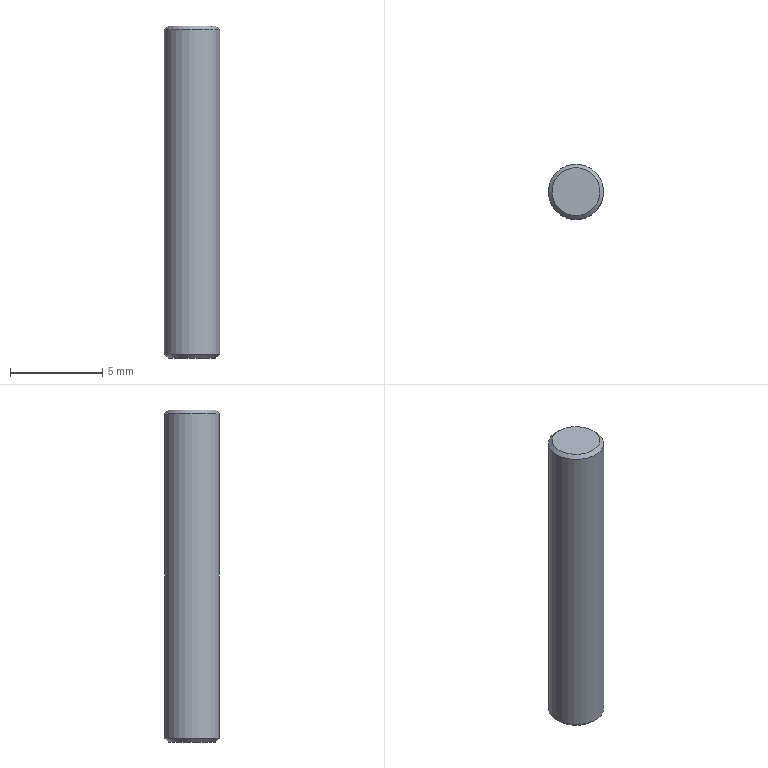Component | NX | GB120-3X20 | 1 solid | 5 faces | box 3 x 3 x 18 mm | volume 127 mm3 | plane 2 | cone 2 | cylinder 1 | commonest cylinder face diameters 3 x1
STEP:
#1=CARTESIAN_POINT('',(0.,0.,0.));
#2=DIRECTION('',(0.,0.,1.));
#3=DIRECTION('',(1.,0.,0.));
#4=AXIS2_PLACEMENT_3D('',#1,#2,#3);
#5=CARTESIAN_POINT('',(23.5,-0.,41.8));
#6=VERTEX_POINT('',#5);
#7=CARTESIAN_POINT('',(22.,-0.,41.8));
#8=DIRECTION('',(0.,0.,-1.));
#9=DIRECTION('',(1.,0.,0.));
#10=AXIS2_PLACEMENT_3D('',#7,#8,#9);
#11=CIRCLE('',#10,1.5);
#12=CARTESIAN_POINT('',(22.,-0.,42.));
#13=DIRECTION('',(0.,0.,-1.));
#14=DIRECTION('',(-1.,0.,0.));
#15=AXIS2_PLACEMENT_3D('',#12,#13,#14);
#16=CYLINDRICAL_SURFACE('',#15,1.5);
#17=CARTESIAN_POINT('',(3.142,0.2));
#18=DIRECTION('',(1.,0.));
#19=VECTOR('',#18,1.);
#20=LINE('',#17,#19);
#21=(GEOMETRIC_REPRESENTATION_CONTEXT(2)PARAMETRIC_REPRESENTATION_CONTEXT()REPRESENTATION_CONTEXT('',''));
#22=DEFINITIONAL_REPRESENTATION('',(#20),#21);
#23=PCURVE('',#16,#22);
#24=CARTESIAN_POINT('',(22.,-0.,42.));
#25=DIRECTION('',(0.,0.,-1.));
#26=DIRECTION('',(-1.,0.,0.));
#27=AXIS2_PLACEMENT_3D('',#24,#25,#26);
#28=CONICAL_SURFACE('',#27,1.3,0.7854);
#29=CARTESIAN_POINT('',(3.142,0.2));
#30=DIRECTION('',(1.,0.));
#31=VECTOR('',#30,1.);
#32=LINE('',#29,#31);
#33=(GEOMETRIC_REPRESENTATION_CONTEXT(2)PARAMETRIC_REPRESENTATION_CONTEXT()REPRESENTATION_CONTEXT('',''));
#34=DEFINITIONAL_REPRESENTATION('',(#32),#33);
#35=PCURVE('',#28,#34);
#36=SURFACE_CURVE('',#11,(#23,#35),.PCURVE_S1.);
#37=EDGE_CURVE('',#6,#6,#36,.T.);
#38=ORIENTED_EDGE('',*,*,#37,.T.);
#39=CARTESIAN_POINT('',(23.5,-0.,24.2));
#40=VERTEX_POINT('',#39);
#41=CARTESIAN_POINT('',(23.5,-0.,41.8));
#42=CARTESIAN_POINT('',(23.5,-0.,24.2));
#43=B_SPLINE_CURVE_WITH_KNOTS('',1,(#41,#42),.UNSPECIFIED.,.F.,.F.,(2,2),(0.2,17.8),.PIECEWISE_BEZIER_KNOTS.);
#44=CARTESIAN_POINT('',(9.425,0.));
#45=DIRECTION('',(0.,1.));
#46=VECTOR('',#45,1.);
#47=LINE('',#44,#46);
#48=(GEOMETRIC_REPRESENTATION_CONTEXT(2)PARAMETRIC_REPRESENTATION_CONTEXT()REPRESENTATION_CONTEXT('',''));
#49=DEFINITIONAL_REPRESENTATION('',(#47),#48);
#50=PCURVE('',#16,#49);
#51=CARTESIAN_POINT('',(3.142,0.));
#52=DIRECTION('',(0.,1.));
#53=VECTOR('',#52,1.);
#54=LINE('',#51,#53);
#55=(GEOMETRIC_REPRESENTATION_CONTEXT(2)PARAMETRIC_REPRESENTATION_CONTEXT()REPRESENTATION_CONTEXT('',''));
#56=DEFINITIONAL_REPRESENTATION('',(#54),#55);
#57=PCURVE('',#16,#56);
#58=SEAM_CURVE('',#43,(#50,#57),.PCURVE_S1.);
#59=EDGE_CURVE('',#6,#40,#58,.T.);
#60=ORIENTED_EDGE('',*,*,#59,.T.);
#61=CARTESIAN_POINT('',(22.,-0.,24.2));
#62=DIRECTION('',(0.,0.,1.));
#63=DIRECTION('',(1.,0.,0.));
#64=AXIS2_PLACEMENT_3D('',#61,#62,#63);
#65=CIRCLE('',#64,1.5);
#66=CARTESIAN_POINT('',(9.425,17.8));
#67=DIRECTION('',(-1.,0.));
#68=VECTOR('',#67,1.);
#69=LINE('',#66,#68);
#70=(GEOMETRIC_REPRESENTATION_CONTEXT(2)PARAMETRIC_REPRESENTATION_CONTEXT()REPRESENTATION_CONTEXT('',''));
#71=DEFINITIONAL_REPRESENTATION('',(#69),#70);
#72=PCURVE('',#16,#71);
#73=CARTESIAN_POINT('',(22.,-0.,24.2));
#74=DIRECTION('',(0.,0.,1.));
#75=DIRECTION('',(1.,0.,0.));
#76=AXIS2_PLACEMENT_3D('',#73,#74,#75);
#77=CONICAL_SURFACE('',#76,1.5,0.7854);
#78=CARTESIAN_POINT('',(0.,0.));
#79=DIRECTION('',(1.,0.));
#80=VECTOR('',#79,1.);
#81=LINE('',#78,#80);
#82=(GEOMETRIC_REPRESENTATION_CONTEXT(2)PARAMETRIC_REPRESENTATION_CONTEXT()REPRESENTATION_CONTEXT('',''));
#83=DEFINITIONAL_REPRESENTATION('',(#81),#82);
#84=PCURVE('',#77,#83);
#85=SURFACE_CURVE('',#65,(#72,#84),.PCURVE_S1.);
#86=EDGE_CURVE('',#40,#40,#85,.T.);
#87=ORIENTED_EDGE('',*,*,#86,.T.);
#88=ORIENTED_EDGE('',*,*,#59,.F.);
#89=EDGE_LOOP('',(#38,#60,#87,#88));
#90=FACE_BOUND('',#89,.T.);
#91=ADVANCED_FACE('',(#90),#16,.T.);
#92=CARTESIAN_POINT('',(23.3,-0.,42.));
#93=VERTEX_POINT('',#92);
#94=CARTESIAN_POINT('',(22.,-0.,42.));
#95=DIRECTION('',(0.,0.,1.));
#96=DIRECTION('',(1.,0.,0.));
#97=AXIS2_PLACEMENT_3D('',#94,#95,#96);
#98=CIRCLE('',#97,1.3);
#99=CARTESIAN_POINT('',(22.,-0.,42.));
#100=DIRECTION('',(0.,0.,1.));
#101=DIRECTION('',(1.,0.,0.));
#102=AXIS2_PLACEMENT_3D('',#99,#100,#101);
#103=PLANE('',#102);
#104=CARTESIAN_POINT('',(0.,0.));
#105=DIRECTION('',(1.,0.));
#106=AXIS2_PLACEMENT_2D('',#104,#105);
#107=CIRCLE('',#106,1.3);
#108=(GEOMETRIC_REPRESENTATION_CONTEXT(2)PARAMETRIC_REPRESENTATION_CONTEXT()REPRESENTATION_CONTEXT('',''));
#109=DEFINITIONAL_REPRESENTATION('',(#107),#108);
#110=PCURVE('',#103,#109);
#111=CARTESIAN_POINT('',(9.425,0.));
#112=DIRECTION('',(-1.,0.));
#113=VECTOR('',#112,1.);
#114=LINE('',#111,#113);
#115=(GEOMETRIC_REPRESENTATION_CONTEXT(2)PARAMETRIC_REPRESENTATION_CONTEXT()REPRESENTATION_CONTEXT('',''));
#116=DEFINITIONAL_REPRESENTATION('',(#114),#115);
#117=PCURVE('',#28,#116);
#118=SURFACE_CURVE('',#98,(#110,#117),.PCURVE_S1.);
#119=EDGE_CURVE('',#93,#93,#118,.T.);
#120=ORIENTED_EDGE('',*,*,#119,.T.);
#121=EDGE_LOOP('',(#120));
#122=FACE_BOUND('',#121,.T.);
#123=ADVANCED_FACE('',(#122),#103,.T.);
#124=CARTESIAN_POINT('',(23.3,-0.,24.));
#125=VERTEX_POINT('',#124);
#126=CARTESIAN_POINT('',(22.,-0.,24.));
#127=DIRECTION('',(0.,0.,-1.));
#128=DIRECTION('',(1.,0.,0.));
#129=AXIS2_PLACEMENT_3D('',#126,#127,#128);
#130=CIRCLE('',#129,1.3);
#131=CARTESIAN_POINT('',(22.,-0.,24.));
#132=DIRECTION('',(0.,0.,1.));
#133=DIRECTION('',(1.,0.,0.));
#134=AXIS2_PLACEMENT_3D('',#131,#132,#133);
#135=PLANE('',#134);
#136=CARTESIAN_POINT('',(1.3,0.));
#137=CARTESIAN_POINT('',(1.3,-2.252));
#138=CARTESIAN_POINT('',(-0.65,-1.126));
#139=CARTESIAN_POINT('',(-2.6,-0.));
#140=CARTESIAN_POINT('',(-0.65,1.126));
#141=CARTESIAN_POINT('',(1.3,2.252));
#142=CARTESIAN_POINT('',(1.3,0.));
#143=(BOUNDED_CURVE()B_SPLINE_CURVE(2,(#136,#137,#138,#139,#140,#141,#142),.UNSPECIFIED.,.T.,.F.)B_SPLINE_CURVE_WITH_KNOTS((1,2,2,2,2,1),(-2.094,0.,2.094,4.189,6.283,8.378),.UNSPECIFIED.)CURVE()GEOMETRIC_REPRESENTATION_ITEM()RATIONAL_B_SPLINE_CURVE((1.,0.5,1.,0.5,1.,0.5,1.))REPRESENTATION_ITEM(''));
#144=(GEOMETRIC_REPRESENTATION_CONTEXT(2)PARAMETRIC_REPRESENTATION_CONTEXT()REPRESENTATION_CONTEXT('',''));
#145=DEFINITIONAL_REPRESENTATION('',(#143),#144);
#146=PCURVE('',#135,#145);
#147=CARTESIAN_POINT('',(6.283,-0.2));
#148=DIRECTION('',(-1.,0.));
#149=VECTOR('',#148,1.);
#150=LINE('',#147,#149);
#151=(GEOMETRIC_REPRESENTATION_CONTEXT(2)PARAMETRIC_REPRESENTATION_CONTEXT()REPRESENTATION_CONTEXT('',''));
#152=DEFINITIONAL_REPRESENTATION('',(#150),#151);
#153=PCURVE('',#77,#152);
#154=SURFACE_CURVE('',#130,(#146,#153),.PCURVE_S1.);
#155=EDGE_CURVE('',#125,#125,#154,.T.);
#156=ORIENTED_EDGE('',*,*,#155,.T.);
#157=EDGE_LOOP('',(#156));
#158=FACE_BOUND('',#157,.T.);
#159=ADVANCED_FACE('',(#158),#135,.F.);
#160=ORIENTED_EDGE('',*,*,#37,.F.);
#161=CARTESIAN_POINT('',(23.3,-0.,42.));
#162=CARTESIAN_POINT('',(23.5,-0.,41.8));
#163=B_SPLINE_CURVE_WITH_KNOTS('',1,(#161,#162),.UNSPECIFIED.,.F.,.F.,(2,2),(0.,0.2828),.PIECEWISE_BEZIER_KNOTS.);
#164=CARTESIAN_POINT('',(3.142,0.));
#165=DIRECTION('',(0.,1.));
#166=VECTOR('',#165,1.);
#167=LINE('',#164,#166);
#168=(GEOMETRIC_REPRESENTATION_CONTEXT(2)PARAMETRIC_REPRESENTATION_CONTEXT()REPRESENTATION_CONTEXT('',''));
#169=DEFINITIONAL_REPRESENTATION('',(#167),#168);
#170=PCURVE('',#28,#169);
#171=CARTESIAN_POINT('',(9.425,0.));
#172=DIRECTION('',(0.,1.));
#173=VECTOR('',#172,1.);
#174=LINE('',#171,#173);
#175=(GEOMETRIC_REPRESENTATION_CONTEXT(2)PARAMETRIC_REPRESENTATION_CONTEXT()REPRESENTATION_CONTEXT('',''));
#176=DEFINITIONAL_REPRESENTATION('',(#174),#175);
#177=PCURVE('',#28,#176);
#178=SEAM_CURVE('',#163,(#170,#177),.PCURVE_S1.);
#179=EDGE_CURVE('',#93,#6,#178,.T.);
#180=ORIENTED_EDGE('',*,*,#179,.F.);
#181=ORIENTED_EDGE('',*,*,#119,.F.);
#182=ORIENTED_EDGE('',*,*,#179,.T.);
#183=EDGE_LOOP('',(#160,#180,#181,#182));
#184=FACE_BOUND('',#183,.T.);
#185=ADVANCED_FACE('',(#184),#28,.T.);
#186=ORIENTED_EDGE('',*,*,#155,.F.);
#187=CARTESIAN_POINT('',(23.3,-0.,24.));
#188=CARTESIAN_POINT('',(23.5,-0.,24.2));
#189=B_SPLINE_CURVE_WITH_KNOTS('',1,(#187,#188),.UNSPECIFIED.,.F.,.F.,(2,2),(-0.2828,0.),.PIECEWISE_BEZIER_KNOTS.);
#190=CARTESIAN_POINT('',(6.283,0.));
#191=DIRECTION('',(0.,1.));
#192=VECTOR('',#191,1.);
#193=LINE('',#190,#192);
#194=(GEOMETRIC_REPRESENTATION_CONTEXT(2)PARAMETRIC_REPRESENTATION_CONTEXT()REPRESENTATION_CONTEXT('',''));
#195=DEFINITIONAL_REPRESENTATION('',(#193),#194);
#196=PCURVE('',#77,#195);
#197=CARTESIAN_POINT('',(0.,0.));
#198=DIRECTION('',(0.,1.));
#199=VECTOR('',#198,1.);
#200=LINE('',#197,#199);
#201=(GEOMETRIC_REPRESENTATION_CONTEXT(2)PARAMETRIC_REPRESENTATION_CONTEXT()REPRESENTATION_CONTEXT('',''));
#202=DEFINITIONAL_REPRESENTATION('',(#200),#201);
#203=PCURVE('',#77,#202);
#204=SEAM_CURVE('',#189,(#196,#203),.PCURVE_S1.);
#205=EDGE_CURVE('',#125,#40,#204,.T.);
#206=ORIENTED_EDGE('',*,*,#205,.T.);
#207=ORIENTED_EDGE('',*,*,#86,.F.);
#208=ORIENTED_EDGE('',*,*,#205,.F.);
#209=EDGE_LOOP('',(#186,#206,#207,#208));
#210=FACE_BOUND('',#209,.T.);
#211=ADVANCED_FACE('',(#210),#77,.T.);
#212=CLOSED_SHELL('',(#91,#123,#159,#185,#211));
#213=MANIFOLD_SOLID_BREP('',#212);
#214=(LENGTH_UNIT()NAMED_UNIT(*)SI_UNIT(.MILLI.,.METRE.));
#215=UNCERTAINTY_MEASURE_WITH_UNIT(LENGTH_MEASURE(0.00001),#214,'','');
#216=(NAMED_UNIT(*)PLANE_ANGLE_UNIT()SI_UNIT($,.RADIAN.));
#217=(NAMED_UNIT(*)SI_UNIT($,.STERADIAN.)SOLID_ANGLE_UNIT());
#218=(GEOMETRIC_REPRESENTATION_CONTEXT(3)GLOBAL_UNCERTAINTY_ASSIGNED_CONTEXT((#215))GLOBAL_UNIT_ASSIGNED_CONTEXT((#214,#216,#217))REPRESENTATION_CONTEXT('',''));
#219=ADVANCED_BREP_SHAPE_REPRESENTATION('',(#4,#213),#218);